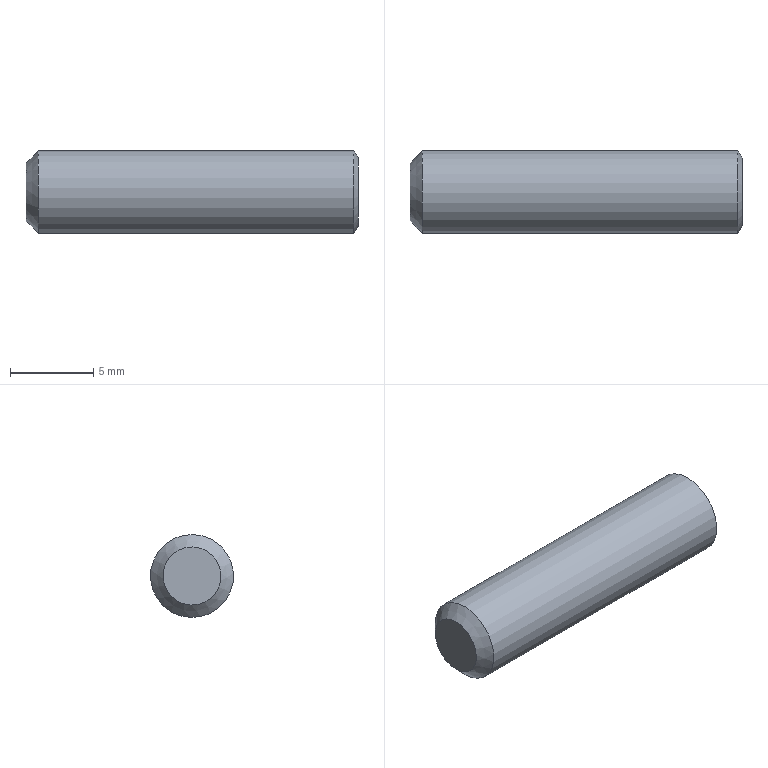Component | NX | LOCK_PIN | 1 solid | 12 faces | box 20 x 5 x 5 mm | volume 372 mm3 | plane 9 | cone 2 | cylinder 1 | commonest cylinder face diameters 5 x1
STEP:
#1=CARTESIAN_POINT('',(0.,0.,0.));
#2=DIRECTION('',(0.,0.,1.));
#3=DIRECTION('',(1.,0.,0.));
#4=AXIS2_PLACEMENT_3D('',#1,#2,#3);
#5=CARTESIAN_POINT('',(-109.177,-1.899,55.707));
#6=VERTEX_POINT('',#5);
#7=CARTESIAN_POINT('',(-109.177,0.,56.491));
#8=DIRECTION('',(1.,0.,0.));
#9=DIRECTION('',(0.,-0.9242,-0.3818));
#10=AXIS2_PLACEMENT_3D('',#7,#8,#9);
#11=CIRCLE('',#10,2.055);
#12=CARTESIAN_POINT('',(-109.177,-1.899,55.707));
#13=DIRECTION('',(-1.,0.,0.));
#14=DIRECTION('',(0.,0.9242,0.3818));
#15=AXIS2_PLACEMENT_3D('',#12,#13,#14);
#16=PLANE('',#15);
#17=CARTESIAN_POINT('',(-0.,0.));
#18=CARTESIAN_POINT('',(-0.,3.559));
#19=CARTESIAN_POINT('',(3.083,1.78));
#20=CARTESIAN_POINT('',(6.165,0.));
#21=CARTESIAN_POINT('',(3.083,-1.78));
#22=CARTESIAN_POINT('',(-0.,-3.559));
#23=CARTESIAN_POINT('',(-0.,0.));
#24=(BOUNDED_CURVE()B_SPLINE_CURVE(2,(#17,#18,#19,#20,#21,#22,#23),.UNSPECIFIED.,.T.,.F.)B_SPLINE_CURVE_WITH_KNOTS((1,2,2,2,2,1),(-2.094,0.,2.094,4.189,6.283,8.378),.UNSPECIFIED.)CURVE()GEOMETRIC_REPRESENTATION_ITEM()RATIONAL_B_SPLINE_CURVE((1.,0.5,1.,0.5,1.,0.5,1.))REPRESENTATION_ITEM(''));
#25=(GEOMETRIC_REPRESENTATION_CONTEXT(2)PARAMETRIC_REPRESENTATION_CONTEXT()REPRESENTATION_CONTEXT('',''));
#26=DEFINITIONAL_REPRESENTATION('',(#24),#25);
#27=PCURVE('',#16,#26);
#28=CARTESIAN_POINT('',(-109.434,0.,56.491));
#29=DIRECTION('',(-1.,0.,0.));
#30=DIRECTION('',(0.,0.9242,0.3818));
#31=AXIS2_PLACEMENT_3D('',#28,#29,#30);
#32=CONICAL_SURFACE('',#31,2.5,1.047);
#33=CARTESIAN_POINT('',(9.425,-0.2569));
#34=DIRECTION('',(-1.,0.));
#35=VECTOR('',#34,1.);
#36=LINE('',#33,#35);
#37=(GEOMETRIC_REPRESENTATION_CONTEXT(2)PARAMETRIC_REPRESENTATION_CONTEXT()REPRESENTATION_CONTEXT('',''));
#38=DEFINITIONAL_REPRESENTATION('',(#36),#37);
#39=PCURVE('',#32,#38);
#40=SURFACE_CURVE('',#11,(#27,#39),.PCURVE_S1.);
#41=EDGE_CURVE('',#6,#6,#40,.T.);
#42=ORIENTED_EDGE('',*,*,#41,.T.);
#43=EDGE_LOOP('',(#42));
#44=FACE_BOUND('',#43,.T.);
#45=CARTESIAN_POINT('',(-109.177,-1.144,57.371));
#46=VERTEX_POINT('',#45);
#47=CARTESIAN_POINT('',(-109.177,0.1897,57.922));
#48=VERTEX_POINT('',#47);
#49=CARTESIAN_POINT('',(-109.177,-1.144,57.371));
#50=DIRECTION('',(0.,0.9242,0.3818));
#51=VECTOR('',#50,1.);
#52=LINE('',#49,#51);
#53=CARTESIAN_POINT('',(1.333,-1.25));
#54=DIRECTION('',(1.,-0.));
#55=VECTOR('',#54,1.);
#56=LINE('',#53,#55);
#57=(GEOMETRIC_REPRESENTATION_CONTEXT(2)PARAMETRIC_REPRESENTATION_CONTEXT()REPRESENTATION_CONTEXT('',''));
#58=DEFINITIONAL_REPRESENTATION('',(#56),#57);
#59=PCURVE('',#16,#58);
#60=CARTESIAN_POINT('',(-112.177,-1.144,57.371));
#61=DIRECTION('',(0.,0.3818,-0.9242));
#62=DIRECTION('',(0.,-0.9242,-0.3818));
#63=AXIS2_PLACEMENT_3D('',#60,#61,#62);
#64=PLANE('',#63);
#65=CARTESIAN_POINT('',(0.,-3.));
#66=DIRECTION('',(-1.,0.));
#67=VECTOR('',#66,1.);
#68=LINE('',#65,#67);
#69=(GEOMETRIC_REPRESENTATION_CONTEXT(2)PARAMETRIC_REPRESENTATION_CONTEXT()REPRESENTATION_CONTEXT('',''));
#70=DEFINITIONAL_REPRESENTATION('',(#68),#69);
#71=PCURVE('',#64,#70);
#72=SURFACE_CURVE('',#52,(#59,#71),.PCURVE_S1.);
#73=EDGE_CURVE('',#46,#48,#72,.T.);
#74=ORIENTED_EDGE('',*,*,#73,.T.);
#75=CARTESIAN_POINT('',(-109.177,1.334,57.043));
#76=VERTEX_POINT('',#75);
#77=CARTESIAN_POINT('',(-109.177,0.1897,57.922));
#78=DIRECTION('',(0.,0.7928,-0.6095));
#79=VECTOR('',#78,1.);
#80=LINE('',#77,#79);
#81=CARTESIAN_POINT('',(2.777,-1.25));
#82=DIRECTION('',(0.5,0.866));
#83=VECTOR('',#82,1.);
#84=LINE('',#81,#83);
#85=(GEOMETRIC_REPRESENTATION_CONTEXT(2)PARAMETRIC_REPRESENTATION_CONTEXT()REPRESENTATION_CONTEXT('',''));
#86=DEFINITIONAL_REPRESENTATION('',(#84),#85);
#87=PCURVE('',#16,#86);
#88=CARTESIAN_POINT('',(-112.177,0.1897,57.922));
#89=DIRECTION('',(0.,-0.6095,-0.7928));
#90=DIRECTION('',(0.,-0.7928,0.6095));
#91=AXIS2_PLACEMENT_3D('',#88,#89,#90);
#92=PLANE('',#91);
#93=CARTESIAN_POINT('',(0.,-3.));
#94=DIRECTION('',(-1.,0.));
#95=VECTOR('',#94,1.);
#96=LINE('',#93,#95);
#97=(GEOMETRIC_REPRESENTATION_CONTEXT(2)PARAMETRIC_REPRESENTATION_CONTEXT()REPRESENTATION_CONTEXT('',''));
#98=DEFINITIONAL_REPRESENTATION('',(#96),#97);
#99=PCURVE('',#92,#98);
#100=SURFACE_CURVE('',#80,(#87,#99),.PCURVE_S1.);
#101=EDGE_CURVE('',#48,#76,#100,.T.);
#102=ORIENTED_EDGE('',*,*,#101,.T.);
#103=CARTESIAN_POINT('',(-109.177,1.144,55.612));
#104=VERTEX_POINT('',#103);
#105=CARTESIAN_POINT('',(-109.177,1.334,57.043));
#106=DIRECTION('',(0.,-0.1314,-0.9913));
#107=VECTOR('',#106,1.);
#108=LINE('',#105,#107);
#109=CARTESIAN_POINT('',(3.498,-0.));
#110=DIRECTION('',(-0.5,0.866));
#111=VECTOR('',#110,1.);
#112=LINE('',#109,#111);
#113=(GEOMETRIC_REPRESENTATION_CONTEXT(2)PARAMETRIC_REPRESENTATION_CONTEXT()REPRESENTATION_CONTEXT('',''));
#114=DEFINITIONAL_REPRESENTATION('',(#112),#113);
#115=PCURVE('',#16,#114);
#116=CARTESIAN_POINT('',(-112.177,1.334,57.043));
#117=DIRECTION('',(0.,-0.9913,0.1314));
#118=DIRECTION('',(0.,0.1314,0.9913));
#119=AXIS2_PLACEMENT_3D('',#116,#117,#118);
#120=PLANE('',#119);
#121=CARTESIAN_POINT('',(0.,-3.));
#122=DIRECTION('',(-1.,0.));
#123=VECTOR('',#122,1.);
#124=LINE('',#121,#123);
#125=(GEOMETRIC_REPRESENTATION_CONTEXT(2)PARAMETRIC_REPRESENTATION_CONTEXT()REPRESENTATION_CONTEXT('',''));
#126=DEFINITIONAL_REPRESENTATION('',(#124),#125);
#127=PCURVE('',#120,#126);
#128=SURFACE_CURVE('',#108,(#115,#127),.PCURVE_S1.);
#129=EDGE_CURVE('',#76,#104,#128,.T.);
#130=ORIENTED_EDGE('',*,*,#129,.T.);
#131=CARTESIAN_POINT('',(-109.177,-0.1897,55.061));
#132=VERTEX_POINT('',#131);
#133=CARTESIAN_POINT('',(-109.177,1.144,55.612));
#134=DIRECTION('',(0.,-0.9242,-0.3818));
#135=VECTOR('',#134,1.);
#136=LINE('',#133,#135);
#137=CARTESIAN_POINT('',(2.777,1.25));
#138=DIRECTION('',(-1.,0.));
#139=VECTOR('',#138,1.);
#140=LINE('',#137,#139);
#141=(GEOMETRIC_REPRESENTATION_CONTEXT(2)PARAMETRIC_REPRESENTATION_CONTEXT()REPRESENTATION_CONTEXT('',''));
#142=DEFINITIONAL_REPRESENTATION('',(#140),#141);
#143=PCURVE('',#16,#142);
#144=CARTESIAN_POINT('',(-112.177,1.144,55.612));
#145=DIRECTION('',(0.,-0.3818,0.9242));
#146=DIRECTION('',(0.,0.9242,0.3818));
#147=AXIS2_PLACEMENT_3D('',#144,#145,#146);
#148=PLANE('',#147);
#149=CARTESIAN_POINT('',(0.,-3.));
#150=DIRECTION('',(-1.,0.));
#151=VECTOR('',#150,1.);
#152=LINE('',#149,#151);
#153=(GEOMETRIC_REPRESENTATION_CONTEXT(2)PARAMETRIC_REPRESENTATION_CONTEXT()REPRESENTATION_CONTEXT('',''));
#154=DEFINITIONAL_REPRESENTATION('',(#152),#153);
#155=PCURVE('',#148,#154);
#156=SURFACE_CURVE('',#136,(#143,#155),.PCURVE_S1.);
#157=EDGE_CURVE('',#104,#132,#156,.T.);
#158=ORIENTED_EDGE('',*,*,#157,.T.);
#159=CARTESIAN_POINT('',(-109.177,-1.334,55.94));
#160=VERTEX_POINT('',#159);
#161=CARTESIAN_POINT('',(-109.177,-0.1897,55.061));
#162=DIRECTION('',(0.,-0.7928,0.6095));
#163=VECTOR('',#162,1.);
#164=LINE('',#161,#163);
#165=CARTESIAN_POINT('',(1.333,1.25));
#166=DIRECTION('',(-0.5,-0.866));
#167=VECTOR('',#166,1.);
#168=LINE('',#165,#167);
#169=(GEOMETRIC_REPRESENTATION_CONTEXT(2)PARAMETRIC_REPRESENTATION_CONTEXT()REPRESENTATION_CONTEXT('',''));
#170=DEFINITIONAL_REPRESENTATION('',(#168),#169);
#171=PCURVE('',#16,#170);
#172=CARTESIAN_POINT('',(-112.177,-0.1897,55.061));
#173=DIRECTION('',(0.,0.6095,0.7928));
#174=DIRECTION('',(0.,0.7928,-0.6095));
#175=AXIS2_PLACEMENT_3D('',#172,#173,#174);
#176=PLANE('',#175);
#177=CARTESIAN_POINT('',(0.,-3.));
#178=DIRECTION('',(-1.,0.));
#179=VECTOR('',#178,1.);
#180=LINE('',#177,#179);
#181=(GEOMETRIC_REPRESENTATION_CONTEXT(2)PARAMETRIC_REPRESENTATION_CONTEXT()REPRESENTATION_CONTEXT('',''));
#182=DEFINITIONAL_REPRESENTATION('',(#180),#181);
#183=PCURVE('',#176,#182);
#184=SURFACE_CURVE('',#164,(#171,#183),.PCURVE_S1.);
#185=EDGE_CURVE('',#132,#160,#184,.T.);
#186=ORIENTED_EDGE('',*,*,#185,.T.);
#187=CARTESIAN_POINT('',(-109.177,-1.334,55.94));
#188=DIRECTION('',(0.,0.1314,0.9913));
#189=VECTOR('',#188,1.);
#190=LINE('',#187,#189);
#191=CARTESIAN_POINT('',(0.6116,-0.));
#192=DIRECTION('',(0.5,-0.866));
#193=VECTOR('',#192,1.);
#194=LINE('',#191,#193);
#195=(GEOMETRIC_REPRESENTATION_CONTEXT(2)PARAMETRIC_REPRESENTATION_CONTEXT()REPRESENTATION_CONTEXT('',''));
#196=DEFINITIONAL_REPRESENTATION('',(#194),#195);
#197=PCURVE('',#16,#196);
#198=CARTESIAN_POINT('',(-112.177,-1.334,55.94));
#199=DIRECTION('',(0.,0.9913,-0.1314));
#200=DIRECTION('',(0.,-0.1314,-0.9913));
#201=AXIS2_PLACEMENT_3D('',#198,#199,#200);
#202=PLANE('',#201);
#203=CARTESIAN_POINT('',(0.,-3.));
#204=DIRECTION('',(-1.,0.));
#205=VECTOR('',#204,1.);
#206=LINE('',#203,#205);
#207=(GEOMETRIC_REPRESENTATION_CONTEXT(2)PARAMETRIC_REPRESENTATION_CONTEXT()REPRESENTATION_CONTEXT('',''));
#208=DEFINITIONAL_REPRESENTATION('',(#206),#207);
#209=PCURVE('',#202,#208);
#210=SURFACE_CURVE('',#190,(#197,#209),.PCURVE_S1.);
#211=EDGE_CURVE('',#160,#46,#210,.T.);
#212=ORIENTED_EDGE('',*,*,#211,.T.);
#213=EDGE_LOOP('',(#74,#102,#130,#158,#186,#212));
#214=FACE_BOUND('',#213,.T.);
#215=ADVANCED_FACE('',(#44,#214),#16,.F.);
#216=CARTESIAN_POINT('',(-129.177,-1.617,55.823));
#217=VERTEX_POINT('',#216);
#218=CARTESIAN_POINT('',(-129.177,0.,56.491));
#219=DIRECTION('',(1.,0.,0.));
#220=DIRECTION('',(0.,-0.9242,-0.3818));
#221=AXIS2_PLACEMENT_3D('',#218,#219,#220);
#222=CIRCLE('',#221,1.75);
#223=CARTESIAN_POINT('',(-129.177,0.,56.491));
#224=DIRECTION('',(1.,0.,0.));
#225=DIRECTION('',(0.,-0.9242,-0.3818));
#226=AXIS2_PLACEMENT_3D('',#223,#224,#225);
#227=PLANE('',#226);
#228=CARTESIAN_POINT('',(0.,-0.));
#229=DIRECTION('',(1.,-0.));
#230=AXIS2_PLACEMENT_2D('',#228,#229);
#231=CIRCLE('',#230,1.75);
#232=(GEOMETRIC_REPRESENTATION_CONTEXT(2)PARAMETRIC_REPRESENTATION_CONTEXT()REPRESENTATION_CONTEXT('',''));
#233=DEFINITIONAL_REPRESENTATION('',(#231),#232);
#234=PCURVE('',#227,#233);
#235=CARTESIAN_POINT('',(-129.177,0.,56.491));
#236=DIRECTION('',(1.,0.,0.));
#237=DIRECTION('',(0.,-0.9242,-0.3818));
#238=AXIS2_PLACEMENT_3D('',#235,#236,#237);
#239=CONICAL_SURFACE('',#238,1.75,0.7854);
#240=CARTESIAN_POINT('',(0.,0.));
#241=DIRECTION('',(1.,0.));
#242=VECTOR('',#241,1.);
#243=LINE('',#240,#242);
#244=(GEOMETRIC_REPRESENTATION_CONTEXT(2)PARAMETRIC_REPRESENTATION_CONTEXT()REPRESENTATION_CONTEXT('',''));
#245=DEFINITIONAL_REPRESENTATION('',(#243),#244);
#246=PCURVE('',#239,#245);
#247=SURFACE_CURVE('',#222,(#234,#246),.PCURVE_S1.);
#248=EDGE_CURVE('',#217,#217,#247,.T.);
#249=ORIENTED_EDGE('',*,*,#248,.F.);
#250=EDGE_LOOP('',(#249));
#251=FACE_BOUND('',#250,.T.);
#252=ADVANCED_FACE('',(#251),#227,.F.);
#253=CARTESIAN_POINT('',(-128.427,-2.311,55.537));
#254=VERTEX_POINT('',#253);
#255=CARTESIAN_POINT('',(-128.427,0.,56.491));
#256=DIRECTION('',(1.,0.,0.));
#257=DIRECTION('',(0.,-0.9242,-0.3818));
#258=AXIS2_PLACEMENT_3D('',#255,#256,#257);
#259=CIRCLE('',#258,2.5);
#260=CARTESIAN_POINT('',(0.,0.75));
#261=DIRECTION('',(1.,0.));
#262=VECTOR('',#261,1.);
#263=LINE('',#260,#262);
#264=(GEOMETRIC_REPRESENTATION_CONTEXT(2)PARAMETRIC_REPRESENTATION_CONTEXT()REPRESENTATION_CONTEXT('',''));
#265=DEFINITIONAL_REPRESENTATION('',(#263),#264);
#266=PCURVE('',#239,#265);
#267=CARTESIAN_POINT('',(-109.177,0.,56.491));
#268=DIRECTION('',(1.,0.,0.));
#269=DIRECTION('',(0.,-0.9242,-0.3818));
#270=AXIS2_PLACEMENT_3D('',#267,#268,#269);
#271=CYLINDRICAL_SURFACE('',#270,2.5);
#272=CARTESIAN_POINT('',(0.,-19.25));
#273=DIRECTION('',(1.,0.));
#274=VECTOR('',#273,1.);
#275=LINE('',#272,#274);
#276=(GEOMETRIC_REPRESENTATION_CONTEXT(2)PARAMETRIC_REPRESENTATION_CONTEXT()REPRESENTATION_CONTEXT('',''));
#277=DEFINITIONAL_REPRESENTATION('',(#275),#276);
#278=PCURVE('',#271,#277);
#279=SURFACE_CURVE('',#259,(#266,#278),.PCURVE_S1.);
#280=EDGE_CURVE('',#254,#254,#279,.T.);
#281=ORIENTED_EDGE('',*,*,#280,.F.);
#282=CARTESIAN_POINT('',(-129.177,-1.617,55.823));
#283=CARTESIAN_POINT('',(-128.427,-2.311,55.537));
#284=B_SPLINE_CURVE_WITH_KNOTS('',1,(#282,#283),.UNSPECIFIED.,.F.,.F.,(2,2),(0.,1.061),.PIECEWISE_BEZIER_KNOTS.);
#285=CARTESIAN_POINT('',(0.,0.));
#286=DIRECTION('',(0.,1.));
#287=VECTOR('',#286,1.);
#288=LINE('',#285,#287);
#289=(GEOMETRIC_REPRESENTATION_CONTEXT(2)PARAMETRIC_REPRESENTATION_CONTEXT()REPRESENTATION_CONTEXT('',''));
#290=DEFINITIONAL_REPRESENTATION('',(#288),#289);
#291=PCURVE('',#239,#290);
#292=CARTESIAN_POINT('',(6.283,0.));
#293=DIRECTION('',(0.,1.));
#294=VECTOR('',#293,1.);
#295=LINE('',#292,#294);
#296=(GEOMETRIC_REPRESENTATION_CONTEXT(2)PARAMETRIC_REPRESENTATION_CONTEXT()REPRESENTATION_CONTEXT('',''));
#297=DEFINITIONAL_REPRESENTATION('',(#295),#296);
#298=PCURVE('',#239,#297);
#299=SEAM_CURVE('',#284,(#291,#298),.PCURVE_S1.);
#300=EDGE_CURVE('',#217,#254,#299,.T.);
#301=ORIENTED_EDGE('',*,*,#300,.F.);
#302=ORIENTED_EDGE('',*,*,#248,.T.);
#303=ORIENTED_EDGE('',*,*,#300,.T.);
#304=EDGE_LOOP('',(#281,#301,#302,#303));
#305=FACE_BOUND('',#304,.T.);
#306=ADVANCED_FACE('',(#305),#239,.T.);
#307=CARTESIAN_POINT('',(-109.434,-2.311,55.537));
#308=VERTEX_POINT('',#307);
#309=CARTESIAN_POINT('',(-109.434,0.,56.491));
#310=DIRECTION('',(1.,0.,0.));
#311=DIRECTION('',(0.,-0.9242,-0.3818));
#312=AXIS2_PLACEMENT_3D('',#309,#310,#311);
#313=CIRCLE('',#312,2.5);
#314=CARTESIAN_POINT('',(0.,-0.2569));
#315=DIRECTION('',(1.,0.));
#316=VECTOR('',#315,1.);
#317=LINE('',#314,#316);
#318=(GEOMETRIC_REPRESENTATION_CONTEXT(2)PARAMETRIC_REPRESENTATION_CONTEXT()REPRESENTATION_CONTEXT('',''));
#319=DEFINITIONAL_REPRESENTATION('',(#317),#318);
#320=PCURVE('',#271,#319);
#321=CARTESIAN_POINT('',(9.425,0.));
#322=DIRECTION('',(-1.,0.));
#323=VECTOR('',#322,1.);
#324=LINE('',#321,#323);
#325=(GEOMETRIC_REPRESENTATION_CONTEXT(2)PARAMETRIC_REPRESENTATION_CONTEXT()REPRESENTATION_CONTEXT('',''));
#326=DEFINITIONAL_REPRESENTATION('',(#324),#325);
#327=PCURVE('',#32,#326);
#328=SURFACE_CURVE('',#313,(#320,#327),.PCURVE_S1.);
#329=EDGE_CURVE('',#308,#308,#328,.T.);
#330=ORIENTED_EDGE('',*,*,#329,.F.);
#331=CARTESIAN_POINT('',(-128.427,-2.311,55.537));
#332=CARTESIAN_POINT('',(-109.434,-2.311,55.537));
#333=B_SPLINE_CURVE_WITH_KNOTS('',1,(#331,#332),.UNSPECIFIED.,.F.,.F.,(2,2),(-19.25,-0.2569),.PIECEWISE_BEZIER_KNOTS.);
#334=CARTESIAN_POINT('',(0.,0.));
#335=DIRECTION('',(0.,1.));
#336=VECTOR('',#335,1.);
#337=LINE('',#334,#336);
#338=(GEOMETRIC_REPRESENTATION_CONTEXT(2)PARAMETRIC_REPRESENTATION_CONTEXT()REPRESENTATION_CONTEXT('',''));
#339=DEFINITIONAL_REPRESENTATION('',(#337),#338);
#340=PCURVE('',#271,#339);
#341=CARTESIAN_POINT('',(6.283,0.));
#342=DIRECTION('',(0.,1.));
#343=VECTOR('',#342,1.);
#344=LINE('',#341,#343);
#345=(GEOMETRIC_REPRESENTATION_CONTEXT(2)PARAMETRIC_REPRESENTATION_CONTEXT()REPRESENTATION_CONTEXT('',''));
#346=DEFINITIONAL_REPRESENTATION('',(#344),#345);
#347=PCURVE('',#271,#346);
#348=SEAM_CURVE('',#333,(#340,#347),.PCURVE_S1.);
#349=EDGE_CURVE('',#254,#308,#348,.T.);
#350=ORIENTED_EDGE('',*,*,#349,.F.);
#351=ORIENTED_EDGE('',*,*,#280,.T.);
#352=ORIENTED_EDGE('',*,*,#349,.T.);
#353=EDGE_LOOP('',(#330,#350,#351,#352));
#354=FACE_BOUND('',#353,.T.);
#355=ADVANCED_FACE('',(#354),#271,.T.);
#356=ORIENTED_EDGE('',*,*,#41,.F.);
#357=CARTESIAN_POINT('',(-109.177,-1.899,55.707));
#358=CARTESIAN_POINT('',(-109.434,-2.311,55.537));
#359=B_SPLINE_CURVE_WITH_KNOTS('',1,(#357,#358),.UNSPECIFIED.,.F.,.F.,(2,2),(-0.5138,0.),.PIECEWISE_BEZIER_KNOTS.);
#360=CARTESIAN_POINT('',(9.425,0.));
#361=DIRECTION('',(0.,1.));
#362=VECTOR('',#361,1.);
#363=LINE('',#360,#362);
#364=(GEOMETRIC_REPRESENTATION_CONTEXT(2)PARAMETRIC_REPRESENTATION_CONTEXT()REPRESENTATION_CONTEXT('',''));
#365=DEFINITIONAL_REPRESENTATION('',(#363),#364);
#366=PCURVE('',#32,#365);
#367=CARTESIAN_POINT('',(3.142,0.));
#368=DIRECTION('',(0.,1.));
#369=VECTOR('',#368,1.);
#370=LINE('',#367,#369);
#371=(GEOMETRIC_REPRESENTATION_CONTEXT(2)PARAMETRIC_REPRESENTATION_CONTEXT()REPRESENTATION_CONTEXT('',''));
#372=DEFINITIONAL_REPRESENTATION('',(#370),#371);
#373=PCURVE('',#32,#372);
#374=SEAM_CURVE('',#359,(#366,#373),.PCURVE_S1.);
#375=EDGE_CURVE('',#6,#308,#374,.T.);
#376=ORIENTED_EDGE('',*,*,#375,.T.);
#377=ORIENTED_EDGE('',*,*,#329,.T.);
#378=ORIENTED_EDGE('',*,*,#375,.F.);
#379=EDGE_LOOP('',(#356,#376,#377,#378));
#380=FACE_BOUND('',#379,.T.);
#381=ADVANCED_FACE('',(#380),#32,.T.);
#382=ORIENTED_EDGE('',*,*,#73,.F.);
#383=CARTESIAN_POINT('',(-112.177,-1.144,57.371));
#384=VERTEX_POINT('',#383);
#385=CARTESIAN_POINT('',(-112.177,-1.144,57.371));
#386=DIRECTION('',(-1.,0.,0.));
#387=VECTOR('',#386,1.);
#388=LINE('',#385,#387);
#389=CARTESIAN_POINT('',(0.,0.));
#390=DIRECTION('',(0.,1.));
#391=VECTOR('',#390,1.);
#392=LINE('',#389,#391);
#393=(GEOMETRIC_REPRESENTATION_CONTEXT(2)PARAMETRIC_REPRESENTATION_CONTEXT()REPRESENTATION_CONTEXT('',''));
#394=DEFINITIONAL_REPRESENTATION('',(#392),#393);
#395=PCURVE('',#64,#394);
#396=CARTESIAN_POINT('',(-1.443,0.));
#397=DIRECTION('',(0.,1.));
#398=VECTOR('',#397,1.);
#399=LINE('',#396,#398);
#400=(GEOMETRIC_REPRESENTATION_CONTEXT(2)PARAMETRIC_REPRESENTATION_CONTEXT()REPRESENTATION_CONTEXT('',''));
#401=DEFINITIONAL_REPRESENTATION('',(#399),#400);
#402=PCURVE('',#202,#401);
#403=SURFACE_CURVE('',#388,(#395,#402),.PCURVE_S1.);
#404=EDGE_CURVE('',#46,#384,#403,.T.);
#405=ORIENTED_EDGE('',*,*,#404,.T.);
#406=CARTESIAN_POINT('',(-112.177,0.1897,57.922));
#407=VERTEX_POINT('',#406);
#408=CARTESIAN_POINT('',(-112.177,-1.144,57.371));
#409=DIRECTION('',(0.,-0.9242,-0.3818));
#410=VECTOR('',#409,1.);
#411=LINE('',#408,#410);
#412=CARTESIAN_POINT('',(0.,0.));
#413=DIRECTION('',(1.,0.));
#414=VECTOR('',#413,1.);
#415=LINE('',#412,#414);
#416=(GEOMETRIC_REPRESENTATION_CONTEXT(2)PARAMETRIC_REPRESENTATION_CONTEXT()REPRESENTATION_CONTEXT('',''));
#417=DEFINITIONAL_REPRESENTATION('',(#415),#416);
#418=PCURVE('',#64,#417);
#419=CARTESIAN_POINT('',(-112.177,0.,56.491));
#420=DIRECTION('',(-1.,0.,0.));
#421=DIRECTION('',(0.,0.9242,0.3818));
#422=AXIS2_PLACEMENT_3D('',#419,#420,#421);
#423=PLANE('',#422);
#424=CARTESIAN_POINT('',(-0.7217,-1.25));
#425=DIRECTION('',(-1.,0.));
#426=VECTOR('',#425,1.);
#427=LINE('',#424,#426);
#428=(GEOMETRIC_REPRESENTATION_CONTEXT(2)PARAMETRIC_REPRESENTATION_CONTEXT()REPRESENTATION_CONTEXT('',''));
#429=DEFINITIONAL_REPRESENTATION('',(#427),#428);
#430=PCURVE('',#423,#429);
#431=SURFACE_CURVE('',#411,(#418,#430),.PCURVE_S1.);
#432=EDGE_CURVE('',#407,#384,#431,.T.);
#433=ORIENTED_EDGE('',*,*,#432,.F.);
#434=CARTESIAN_POINT('',(-112.177,0.1897,57.922));
#435=DIRECTION('',(-1.,0.,0.));
#436=VECTOR('',#435,1.);
#437=LINE('',#434,#436);
#438=CARTESIAN_POINT('',(-1.443,0.));
#439=DIRECTION('',(0.,1.));
#440=VECTOR('',#439,1.);
#441=LINE('',#438,#440);
#442=(GEOMETRIC_REPRESENTATION_CONTEXT(2)PARAMETRIC_REPRESENTATION_CONTEXT()REPRESENTATION_CONTEXT('',''));
#443=DEFINITIONAL_REPRESENTATION('',(#441),#442);
#444=PCURVE('',#64,#443);
#445=CARTESIAN_POINT('',(0.,0.));
#446=DIRECTION('',(0.,1.));
#447=VECTOR('',#446,1.);
#448=LINE('',#445,#447);
#449=(GEOMETRIC_REPRESENTATION_CONTEXT(2)PARAMETRIC_REPRESENTATION_CONTEXT()REPRESENTATION_CONTEXT('',''));
#450=DEFINITIONAL_REPRESENTATION('',(#448),#449);
#451=PCURVE('',#92,#450);
#452=SURFACE_CURVE('',#437,(#444,#451),.PCURVE_S1.);
#453=EDGE_CURVE('',#48,#407,#452,.T.);
#454=ORIENTED_EDGE('',*,*,#453,.F.);
#455=EDGE_LOOP('',(#382,#405,#433,#454));
#456=FACE_BOUND('',#455,.T.);
#457=ADVANCED_FACE('',(#456),#64,.T.);
#458=ORIENTED_EDGE('',*,*,#101,.F.);
#459=ORIENTED_EDGE('',*,*,#453,.T.);
#460=CARTESIAN_POINT('',(-112.177,1.334,57.043));
#461=VERTEX_POINT('',#460);
#462=CARTESIAN_POINT('',(-112.177,0.1897,57.922));
#463=DIRECTION('',(0.,-0.7928,0.6095));
#464=VECTOR('',#463,1.);
#465=LINE('',#462,#464);
#466=CARTESIAN_POINT('',(0.,0.));
#467=DIRECTION('',(1.,0.));
#468=VECTOR('',#467,1.);
#469=LINE('',#466,#468);
#470=(GEOMETRIC_REPRESENTATION_CONTEXT(2)PARAMETRIC_REPRESENTATION_CONTEXT()REPRESENTATION_CONTEXT('',''));
#471=DEFINITIONAL_REPRESENTATION('',(#469),#470);
#472=PCURVE('',#92,#471);
#473=CARTESIAN_POINT('',(0.7217,-1.25));
#474=DIRECTION('',(-0.5,-0.866));
#475=VECTOR('',#474,1.);
#476=LINE('',#473,#475);
#477=(GEOMETRIC_REPRESENTATION_CONTEXT(2)PARAMETRIC_REPRESENTATION_CONTEXT()REPRESENTATION_CONTEXT('',''));
#478=DEFINITIONAL_REPRESENTATION('',(#476),#477);
#479=PCURVE('',#423,#478);
#480=SURFACE_CURVE('',#465,(#472,#479),.PCURVE_S1.);
#481=EDGE_CURVE('',#461,#407,#480,.T.);
#482=ORIENTED_EDGE('',*,*,#481,.F.);
#483=CARTESIAN_POINT('',(-112.177,1.334,57.043));
#484=DIRECTION('',(-1.,0.,0.));
#485=VECTOR('',#484,1.);
#486=LINE('',#483,#485);
#487=CARTESIAN_POINT('',(-1.443,0.));
#488=DIRECTION('',(0.,1.));
#489=VECTOR('',#488,1.);
#490=LINE('',#487,#489);
#491=(GEOMETRIC_REPRESENTATION_CONTEXT(2)PARAMETRIC_REPRESENTATION_CONTEXT()REPRESENTATION_CONTEXT('',''));
#492=DEFINITIONAL_REPRESENTATION('',(#490),#491);
#493=PCURVE('',#92,#492);
#494=CARTESIAN_POINT('',(0.,0.));
#495=DIRECTION('',(0.,1.));
#496=VECTOR('',#495,1.);
#497=LINE('',#494,#496);
#498=(GEOMETRIC_REPRESENTATION_CONTEXT(2)PARAMETRIC_REPRESENTATION_CONTEXT()REPRESENTATION_CONTEXT('',''));
#499=DEFINITIONAL_REPRESENTATION('',(#497),#498);
#500=PCURVE('',#120,#499);
#501=SURFACE_CURVE('',#486,(#493,#500),.PCURVE_S1.);
#502=EDGE_CURVE('',#76,#461,#501,.T.);
#503=ORIENTED_EDGE('',*,*,#502,.F.);
#504=EDGE_LOOP('',(#458,#459,#482,#503));
#505=FACE_BOUND('',#504,.T.);
#506=ADVANCED_FACE('',(#505),#92,.T.);
#507=ORIENTED_EDGE('',*,*,#129,.F.);
#508=ORIENTED_EDGE('',*,*,#502,.T.);
#509=CARTESIAN_POINT('',(-112.177,1.144,55.612));
#510=VERTEX_POINT('',#509);
#511=CARTESIAN_POINT('',(-112.177,1.334,57.043));
#512=DIRECTION('',(0.,0.1314,0.9913));
#513=VECTOR('',#512,1.);
#514=LINE('',#511,#513);
#515=CARTESIAN_POINT('',(0.,0.));
#516=DIRECTION('',(1.,0.));
#517=VECTOR('',#516,1.);
#518=LINE('',#515,#517);
#519=(GEOMETRIC_REPRESENTATION_CONTEXT(2)PARAMETRIC_REPRESENTATION_CONTEXT()REPRESENTATION_CONTEXT('',''));
#520=DEFINITIONAL_REPRESENTATION('',(#518),#519);
#521=PCURVE('',#120,#520);
#522=CARTESIAN_POINT('',(1.443,-0.));
#523=DIRECTION('',(0.5,-0.866));
#524=VECTOR('',#523,1.);
#525=LINE('',#522,#524);
#526=(GEOMETRIC_REPRESENTATION_CONTEXT(2)PARAMETRIC_REPRESENTATION_CONTEXT()REPRESENTATION_CONTEXT('',''));
#527=DEFINITIONAL_REPRESENTATION('',(#525),#526);
#528=PCURVE('',#423,#527);
#529=SURFACE_CURVE('',#514,(#521,#528),.PCURVE_S1.);
#530=EDGE_CURVE('',#510,#461,#529,.T.);
#531=ORIENTED_EDGE('',*,*,#530,.F.);
#532=CARTESIAN_POINT('',(-112.177,1.144,55.612));
#533=DIRECTION('',(-1.,0.,0.));
#534=VECTOR('',#533,1.);
#535=LINE('',#532,#534);
#536=CARTESIAN_POINT('',(-1.443,0.));
#537=DIRECTION('',(0.,1.));
#538=VECTOR('',#537,1.);
#539=LINE('',#536,#538);
#540=(GEOMETRIC_REPRESENTATION_CONTEXT(2)PARAMETRIC_REPRESENTATION_CONTEXT()REPRESENTATION_CONTEXT('',''));
#541=DEFINITIONAL_REPRESENTATION('',(#539),#540);
#542=PCURVE('',#120,#541);
#543=CARTESIAN_POINT('',(0.,0.));
#544=DIRECTION('',(0.,1.));
#545=VECTOR('',#544,1.);
#546=LINE('',#543,#545);
#547=(GEOMETRIC_REPRESENTATION_CONTEXT(2)PARAMETRIC_REPRESENTATION_CONTEXT()REPRESENTATION_CONTEXT('',''));
#548=DEFINITIONAL_REPRESENTATION('',(#546),#547);
#549=PCURVE('',#148,#548);
#550=SURFACE_CURVE('',#535,(#542,#549),.PCURVE_S1.);
#551=EDGE_CURVE('',#104,#510,#550,.T.);
#552=ORIENTED_EDGE('',*,*,#551,.F.);
#553=EDGE_LOOP('',(#507,#508,#531,#552));
#554=FACE_BOUND('',#553,.T.);
#555=ADVANCED_FACE('',(#554),#120,.T.);
#556=ORIENTED_EDGE('',*,*,#157,.F.);
#557=ORIENTED_EDGE('',*,*,#551,.T.);
#558=CARTESIAN_POINT('',(-112.177,-0.1897,55.061));
#559=VERTEX_POINT('',#558);
#560=CARTESIAN_POINT('',(-112.177,1.144,55.612));
#561=DIRECTION('',(0.,0.9242,0.3818));
#562=VECTOR('',#561,1.);
#563=LINE('',#560,#562);
#564=CARTESIAN_POINT('',(0.,0.));
#565=DIRECTION('',(1.,0.));
#566=VECTOR('',#565,1.);
#567=LINE('',#564,#566);
#568=(GEOMETRIC_REPRESENTATION_CONTEXT(2)PARAMETRIC_REPRESENTATION_CONTEXT()REPRESENTATION_CONTEXT('',''));
#569=DEFINITIONAL_REPRESENTATION('',(#567),#568);
#570=PCURVE('',#148,#569);
#571=CARTESIAN_POINT('',(0.7217,1.25));
#572=DIRECTION('',(1.,-0.));
#573=VECTOR('',#572,1.);
#574=LINE('',#571,#573);
#575=(GEOMETRIC_REPRESENTATION_CONTEXT(2)PARAMETRIC_REPRESENTATION_CONTEXT()REPRESENTATION_CONTEXT('',''));
#576=DEFINITIONAL_REPRESENTATION('',(#574),#575);
#577=PCURVE('',#423,#576);
#578=SURFACE_CURVE('',#563,(#570,#577),.PCURVE_S1.);
#579=EDGE_CURVE('',#559,#510,#578,.T.);
#580=ORIENTED_EDGE('',*,*,#579,.F.);
#581=CARTESIAN_POINT('',(-112.177,-0.1897,55.061));
#582=DIRECTION('',(-1.,0.,0.));
#583=VECTOR('',#582,1.);
#584=LINE('',#581,#583);
#585=CARTESIAN_POINT('',(-1.443,0.));
#586=DIRECTION('',(0.,1.));
#587=VECTOR('',#586,1.);
#588=LINE('',#585,#587);
#589=(GEOMETRIC_REPRESENTATION_CONTEXT(2)PARAMETRIC_REPRESENTATION_CONTEXT()REPRESENTATION_CONTEXT('',''));
#590=DEFINITIONAL_REPRESENTATION('',(#588),#589);
#591=PCURVE('',#148,#590);
#592=CARTESIAN_POINT('',(0.,0.));
#593=DIRECTION('',(0.,1.));
#594=VECTOR('',#593,1.);
#595=LINE('',#592,#594);
#596=(GEOMETRIC_REPRESENTATION_CONTEXT(2)PARAMETRIC_REPRESENTATION_CONTEXT()REPRESENTATION_CONTEXT('',''));
#597=DEFINITIONAL_REPRESENTATION('',(#595),#596);
#598=PCURVE('',#176,#597);
#599=SURFACE_CURVE('',#584,(#591,#598),.PCURVE_S1.);
#600=EDGE_CURVE('',#132,#559,#599,.T.);
#601=ORIENTED_EDGE('',*,*,#600,.F.);
#602=EDGE_LOOP('',(#556,#557,#580,#601));
#603=FACE_BOUND('',#602,.T.);
#604=ADVANCED_FACE('',(#603),#148,.T.);
#605=ORIENTED_EDGE('',*,*,#185,.F.);
#606=ORIENTED_EDGE('',*,*,#600,.T.);
#607=CARTESIAN_POINT('',(-112.177,-1.334,55.94));
#608=VERTEX_POINT('',#607);
#609=CARTESIAN_POINT('',(-112.177,-0.1897,55.061));
#610=DIRECTION('',(0.,0.7928,-0.6095));
#611=VECTOR('',#610,1.);
#612=LINE('',#609,#611);
#613=CARTESIAN_POINT('',(0.,0.));
#614=DIRECTION('',(1.,0.));
#615=VECTOR('',#614,1.);
#616=LINE('',#613,#615);
#617=(GEOMETRIC_REPRESENTATION_CONTEXT(2)PARAMETRIC_REPRESENTATION_CONTEXT()REPRESENTATION_CONTEXT('',''));
#618=DEFINITIONAL_REPRESENTATION('',(#616),#617);
#619=PCURVE('',#176,#618);
#620=CARTESIAN_POINT('',(-0.7217,1.25));
#621=DIRECTION('',(0.5,0.866));
#622=VECTOR('',#621,1.);
#623=LINE('',#620,#622);
#624=(GEOMETRIC_REPRESENTATION_CONTEXT(2)PARAMETRIC_REPRESENTATION_CONTEXT()REPRESENTATION_CONTEXT('',''));
#625=DEFINITIONAL_REPRESENTATION('',(#623),#624);
#626=PCURVE('',#423,#625);
#627=SURFACE_CURVE('',#612,(#619,#626),.PCURVE_S1.);
#628=EDGE_CURVE('',#608,#559,#627,.T.);
#629=ORIENTED_EDGE('',*,*,#628,.F.);
#630=CARTESIAN_POINT('',(-112.177,-1.334,55.94));
#631=DIRECTION('',(-1.,0.,0.));
#632=VECTOR('',#631,1.);
#633=LINE('',#630,#632);
#634=CARTESIAN_POINT('',(-1.443,0.));
#635=DIRECTION('',(0.,1.));
#636=VECTOR('',#635,1.);
#637=LINE('',#634,#636);
#638=(GEOMETRIC_REPRESENTATION_CONTEXT(2)PARAMETRIC_REPRESENTATION_CONTEXT()REPRESENTATION_CONTEXT('',''));
#639=DEFINITIONAL_REPRESENTATION('',(#637),#638);
#640=PCURVE('',#176,#639);
#641=CARTESIAN_POINT('',(0.,0.));
#642=DIRECTION('',(0.,1.));
#643=VECTOR('',#642,1.);
#644=LINE('',#641,#643);
#645=(GEOMETRIC_REPRESENTATION_CONTEXT(2)PARAMETRIC_REPRESENTATION_CONTEXT()REPRESENTATION_CONTEXT('',''));
#646=DEFINITIONAL_REPRESENTATION('',(#644),#645);
#647=PCURVE('',#202,#646);
#648=SURFACE_CURVE('',#633,(#640,#647),.PCURVE_S1.);
#649=EDGE_CURVE('',#160,#608,#648,.T.);
#650=ORIENTED_EDGE('',*,*,#649,.F.);
#651=EDGE_LOOP('',(#605,#606,#629,#650));
#652=FACE_BOUND('',#651,.T.);
#653=ADVANCED_FACE('',(#652),#176,.T.);
#654=ORIENTED_EDGE('',*,*,#211,.F.);
#655=ORIENTED_EDGE('',*,*,#649,.T.);
#656=CARTESIAN_POINT('',(-112.177,-1.334,55.94));
#657=DIRECTION('',(0.,-0.1314,-0.9913));
#658=VECTOR('',#657,1.);
#659=LINE('',#656,#658);
#660=CARTESIAN_POINT('',(0.,0.));
#661=DIRECTION('',(1.,0.));
#662=VECTOR('',#661,1.);
#663=LINE('',#660,#662);
#664=(GEOMETRIC_REPRESENTATION_CONTEXT(2)PARAMETRIC_REPRESENTATION_CONTEXT()REPRESENTATION_CONTEXT('',''));
#665=DEFINITIONAL_REPRESENTATION('',(#663),#664);
#666=PCURVE('',#202,#665);
#667=CARTESIAN_POINT('',(-1.443,-0.));
#668=DIRECTION('',(-0.5,0.866));
#669=VECTOR('',#668,1.);
#670=LINE('',#667,#669);
#671=(GEOMETRIC_REPRESENTATION_CONTEXT(2)PARAMETRIC_REPRESENTATION_CONTEXT()REPRESENTATION_CONTEXT('',''));
#672=DEFINITIONAL_REPRESENTATION('',(#670),#671);
#673=PCURVE('',#423,#672);
#674=SURFACE_CURVE('',#659,(#666,#673),.PCURVE_S1.);
#675=EDGE_CURVE('',#384,#608,#674,.T.);
#676=ORIENTED_EDGE('',*,*,#675,.F.);
#677=ORIENTED_EDGE('',*,*,#404,.F.);
#678=EDGE_LOOP('',(#654,#655,#676,#677));
#679=FACE_BOUND('',#678,.T.);
#680=ADVANCED_FACE('',(#679),#202,.T.);
#681=ORIENTED_EDGE('',*,*,#432,.T.);
#682=ORIENTED_EDGE('',*,*,#675,.T.);
#683=ORIENTED_EDGE('',*,*,#628,.T.);
#684=ORIENTED_EDGE('',*,*,#579,.T.);
#685=ORIENTED_EDGE('',*,*,#530,.T.);
#686=ORIENTED_EDGE('',*,*,#481,.T.);
#687=EDGE_LOOP('',(#681,#682,#683,#684,#685,#686));
#688=FACE_BOUND('',#687,.T.);
#689=ADVANCED_FACE('',(#688),#423,.F.);
#690=CLOSED_SHELL('',(#215,#252,#306,#355,#381,#457,#506,#555,#604,#653,#680,#689));
#691=MANIFOLD_SOLID_BREP('',#690);
#692=(LENGTH_UNIT()NAMED_UNIT(*)SI_UNIT(.MILLI.,.METRE.));
#693=UNCERTAINTY_MEASURE_WITH_UNIT(LENGTH_MEASURE(0.000002),#692,'','');
#694=(NAMED_UNIT(*)PLANE_ANGLE_UNIT()SI_UNIT($,.RADIAN.));
#695=(NAMED_UNIT(*)SI_UNIT($,.STERADIAN.)SOLID_ANGLE_UNIT());
#696=(GEOMETRIC_REPRESENTATION_CONTEXT(3)GLOBAL_UNCERTAINTY_ASSIGNED_CONTEXT((#693))GLOBAL_UNIT_ASSIGNED_CONTEXT((#692,#694,#695))REPRESENTATION_CONTEXT('',''));
#697=ADVANCED_BREP_SHAPE_REPRESENTATION('',(#4,#691),#696);